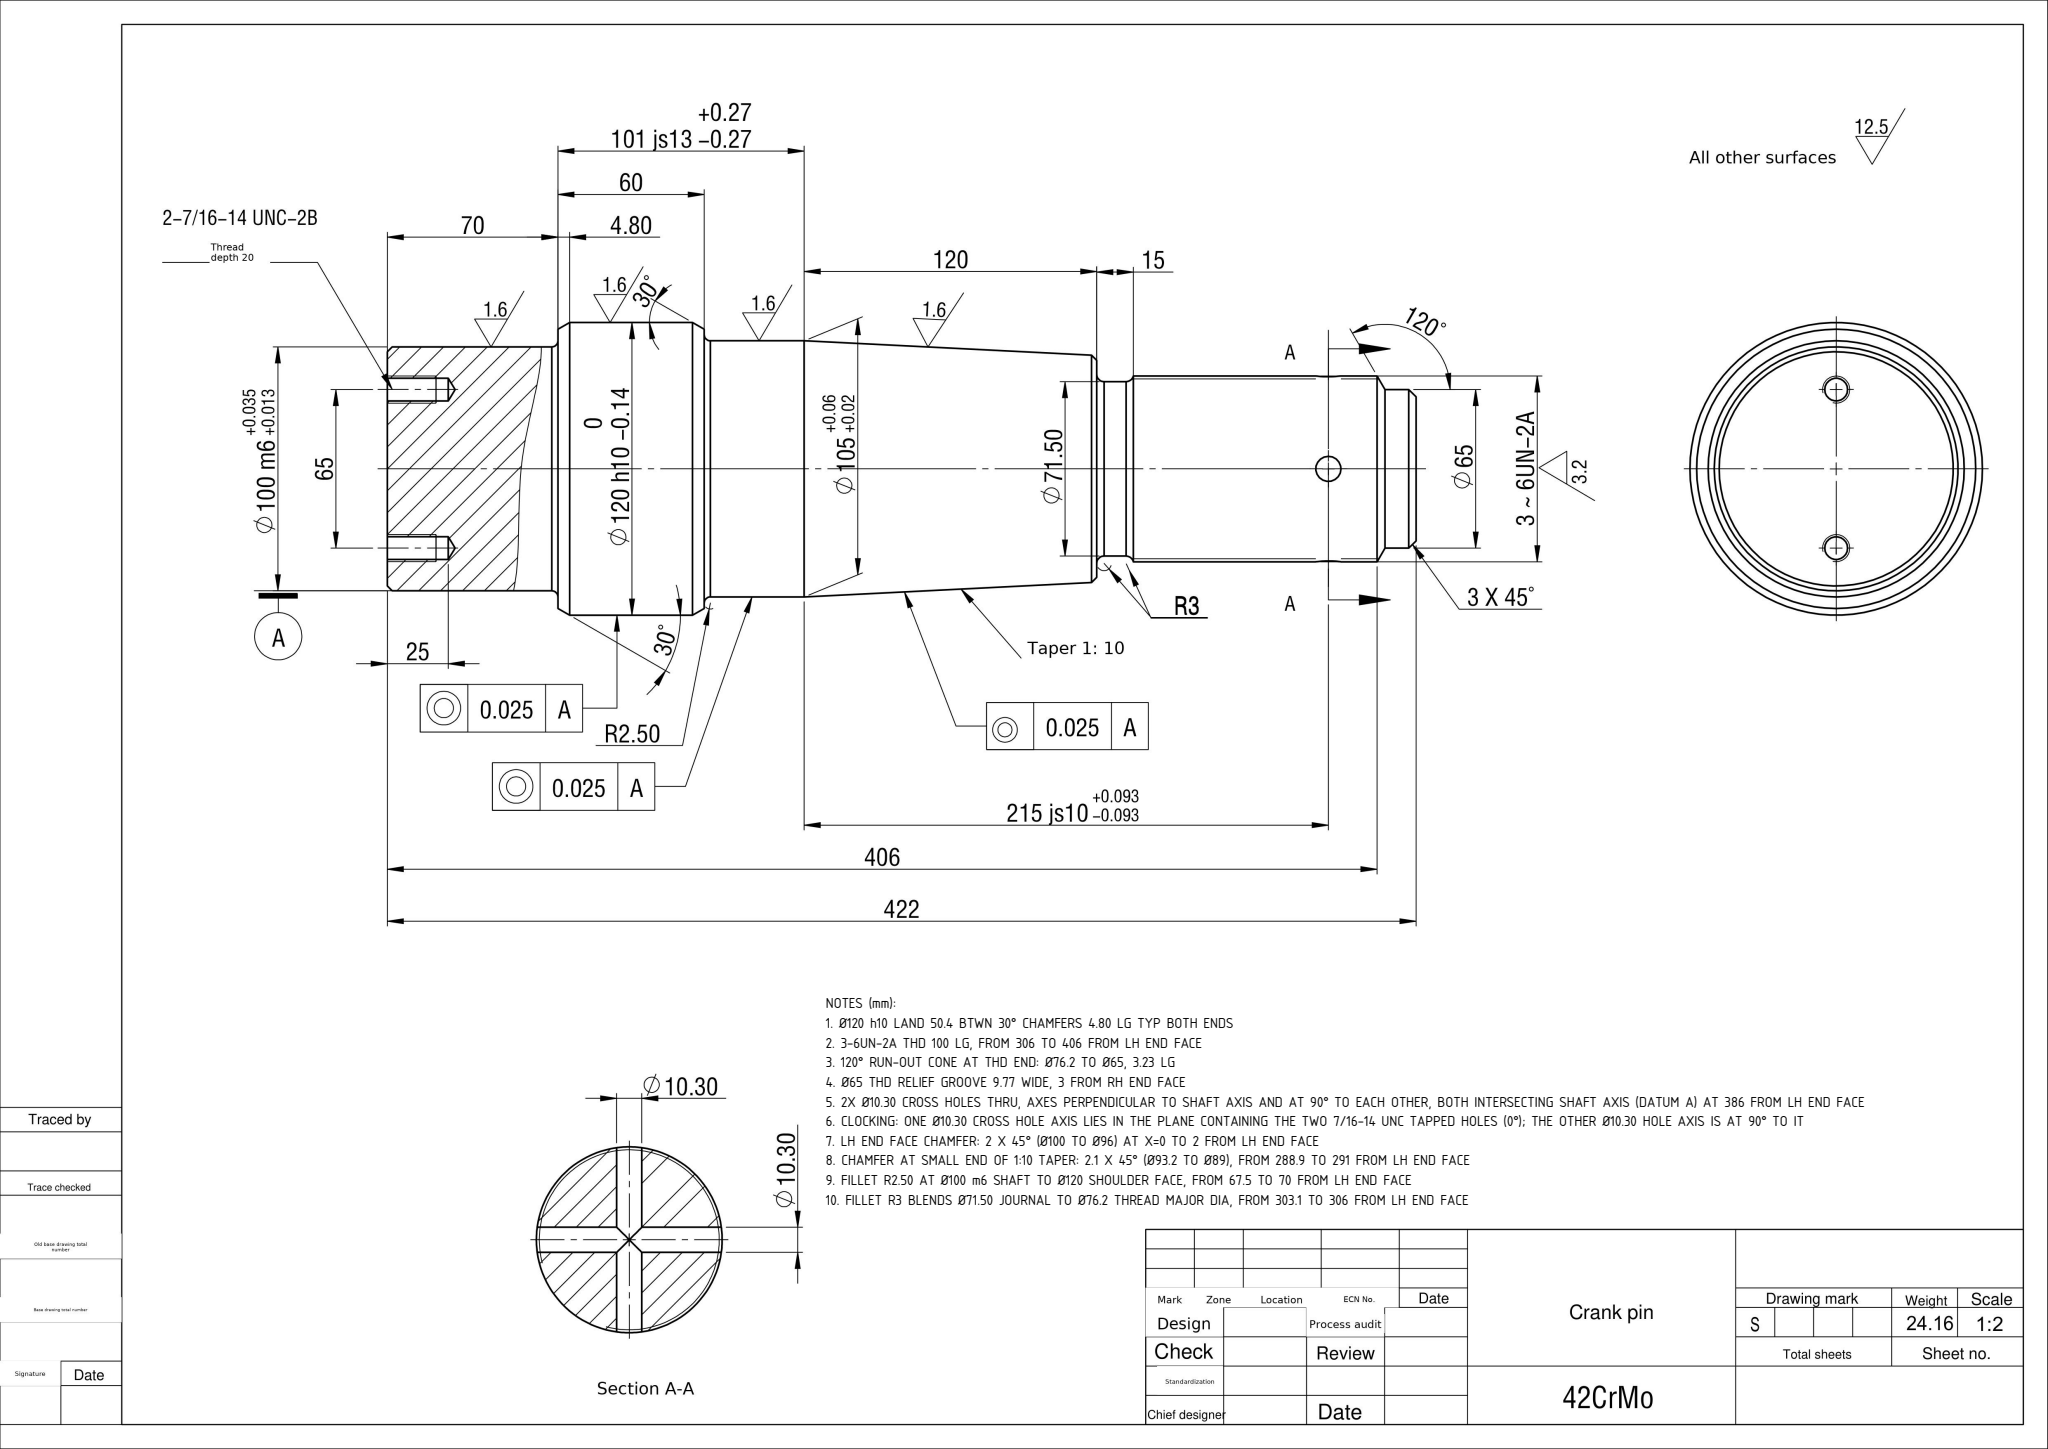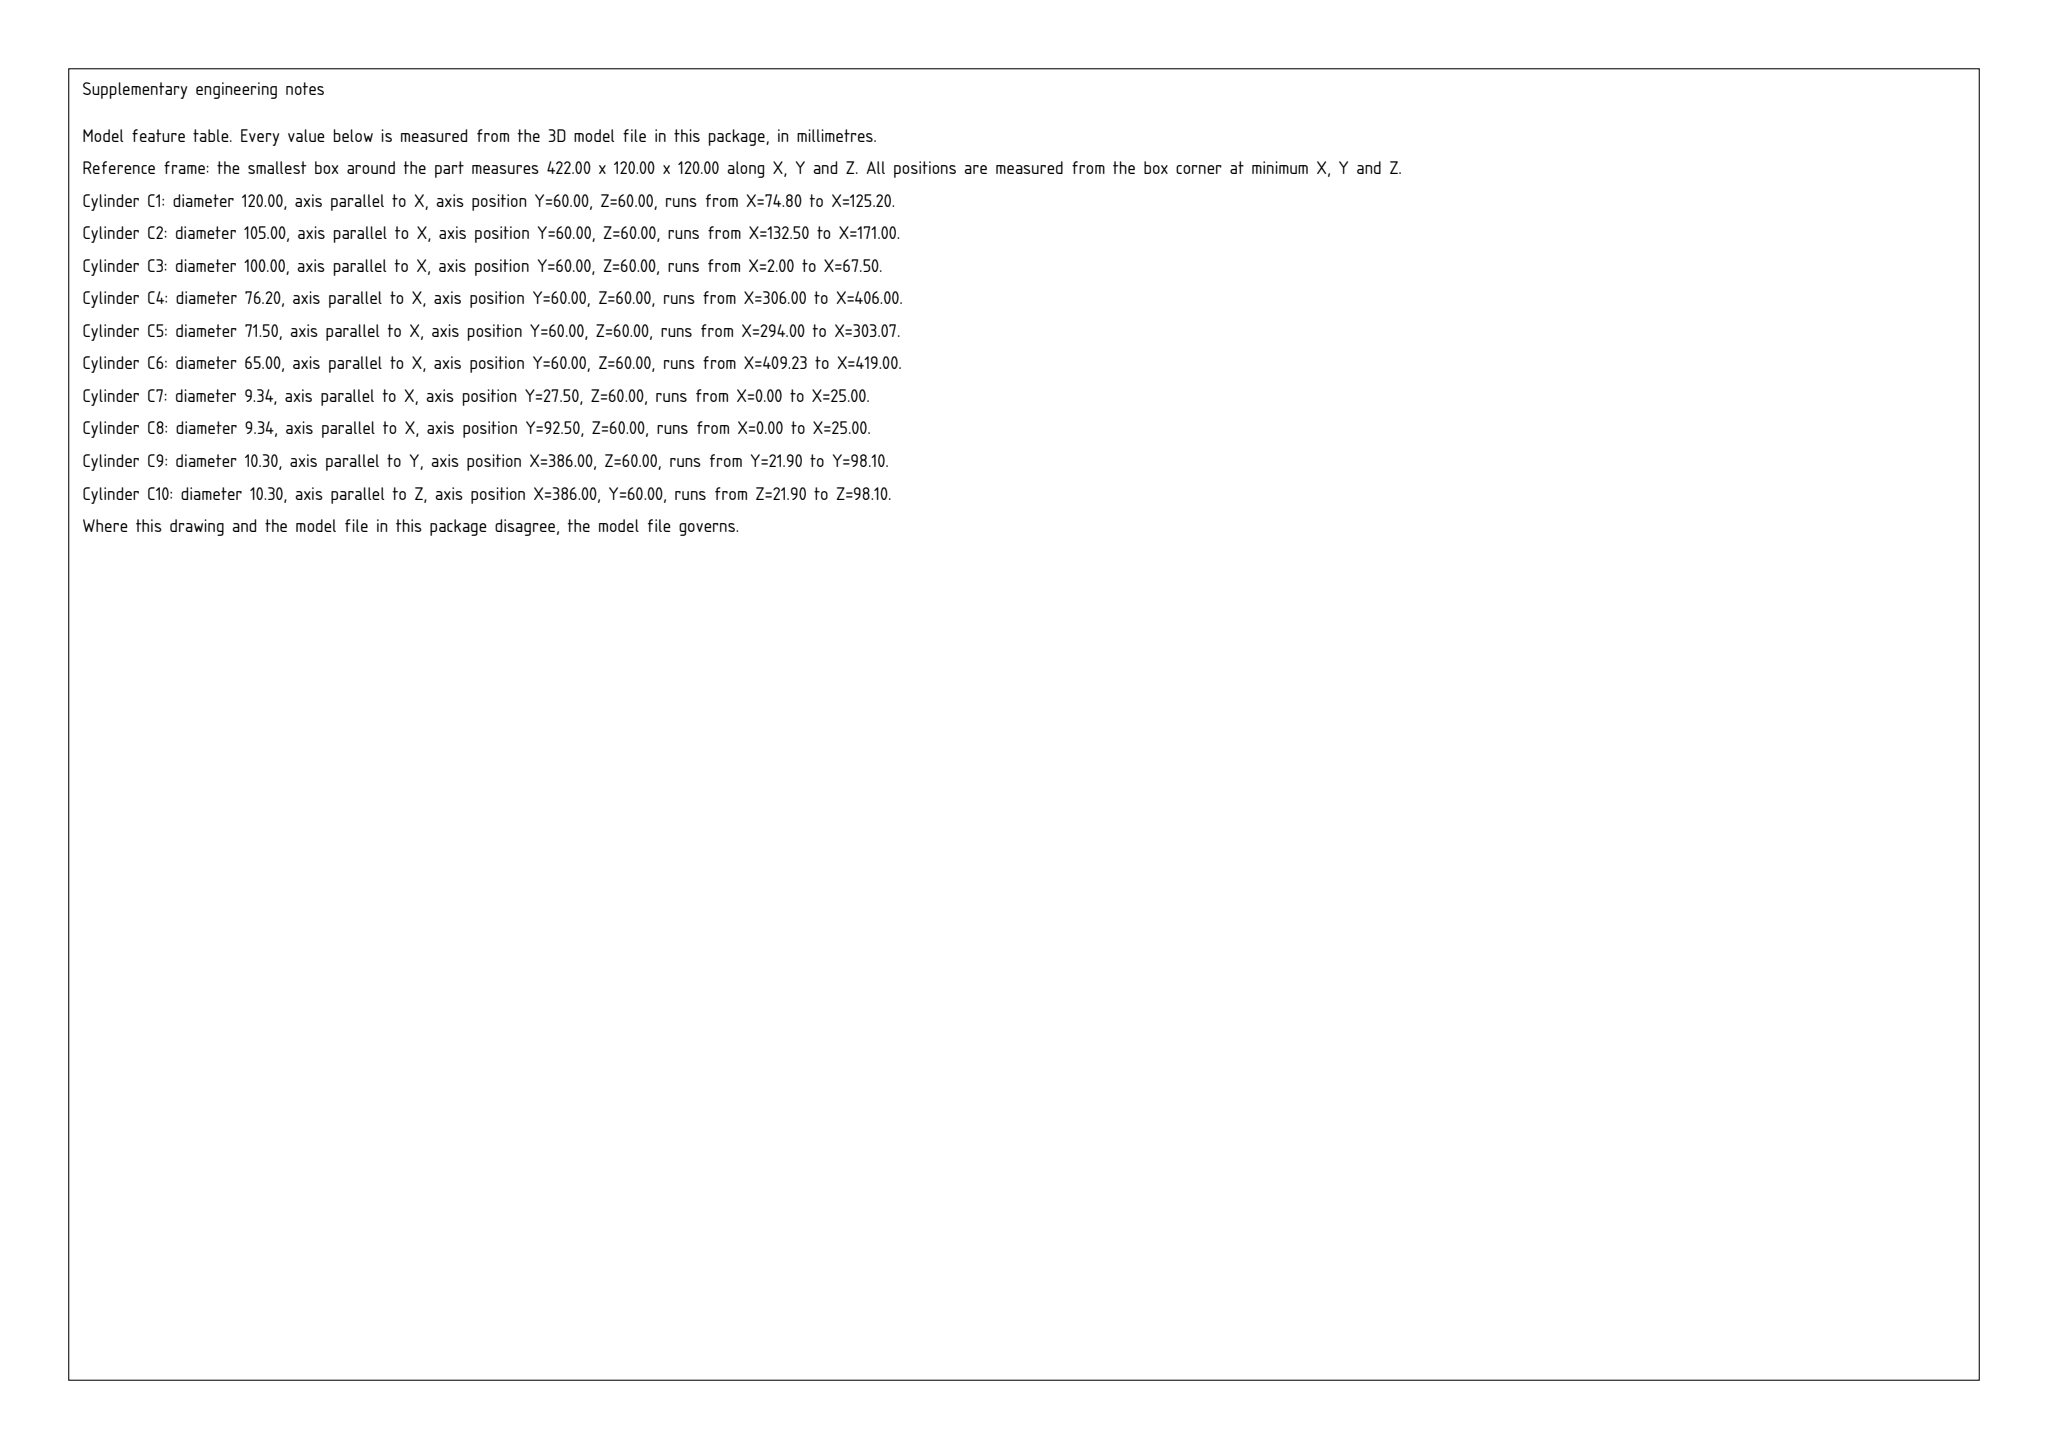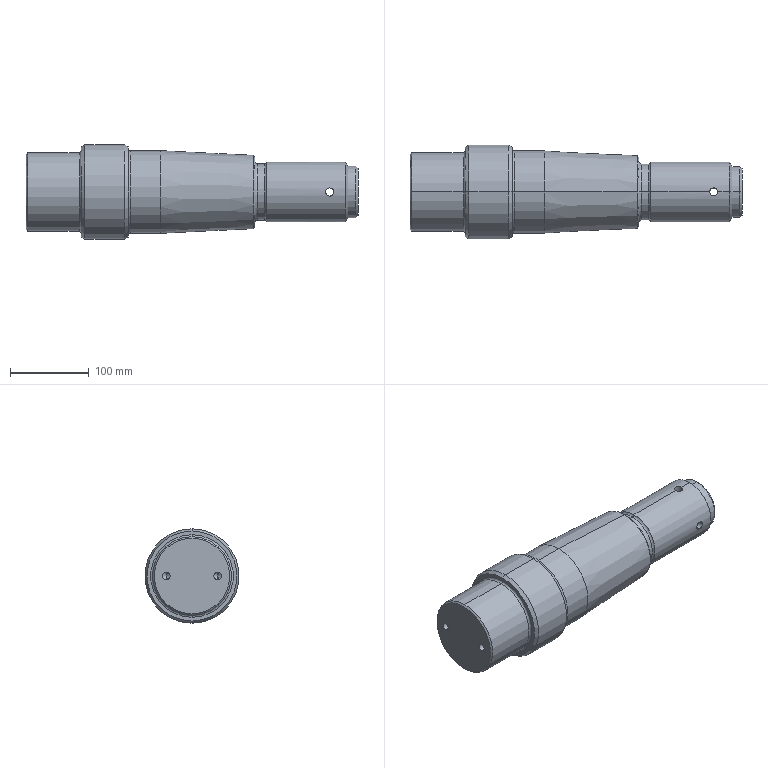Part | SolidWorks | mm | 1 solid | 55 faces | box 422 x 120 x 120 mm | volume 3058705 mm3 | cylinder 24 | cone 18 | torus 8 | plane 5 | commonest cylinder face diameters 10.3 x8 9.347 x4 65 x2 76.2 x2 71.5 x2 105 x2 120 x2 100 x2
Drawing notes:
Ø120 h10 LAND 50.4 BTWN 30° CHAMFERS 4.80 LG TYP BOTH ENDS | from the solid: 60° incl cone ref Ø120/Ø114.457; Ø120 cyl 50.4 = 60 - 2 x 4.80, boss x=70 to 130
3-6UN-2A THD 100 LG, FROM 306 TO 406 FROM LH END FACE | from the solid: Ø76.2 cyl, axis x, length 100, spans x=306 (end of 15 neck) to x=406; bbox x=0 at LH end face
120° RUN-OUT CONE AT THD END: Ø76.2 TO Ø65, 3.23 LG | from the solid: cone incl angle 120°, ref dia 65, joins Ø76.2 thd at x=406 to Ø65 groove at x=409.23
Ø65 THD RELIEF GROOVE 9.77 WIDE, 3 FROM RH END FACE | from the solid: Ø65 cyl length 9.77 (x=409.23 to 419), followed by 90° cone ref Ø65 (3x45 chamfer) to end face x=422
2X Ø10.30 CROSS HOLES THRU, AXES PERPENDICULAR TO SHAFT AXIS AND AT 90° TO EACH OTHER, BOTH INTERSECTING SHAFT AXIS (DATUM A) AT 386 FROM LH END FACE | from the solid: cylinders hole/bore Ø10.3 on y axis at [386,-,60] and Ø10.3 on z axis at [386,60,-], both spanning 21.9 to 98.1 (full 120 width)
CLOCKING: ONE Ø10.30 CROSS HOLE AXIS LIES IN THE PLANE CONTAINING THE TWO 7/16-14 UNC TAPPED HOLES (0°); THE OTHER Ø10.30 HOLE AXIS IS AT 90° TO IT | from the solid: tapped-hole cylinders Ø9.35 on x axis at y=27.5 and y=92.5, z=60 (line parallel to Y); Ø10.3 hole axes are along Y and along Z
LH END FACE CHAMFER: 2 X 45° (Ø100 TO Ø96) AT X=0 TO 2 FROM LH END FACE | from the solid: axis_planes x=0 extent y/z 12.0-108.0 (Ø96 face) with cylinder Ø100 starting at x=2.0
CHAMFER AT SMALL END OF 1:10 TAPER: 2.1 X 45° (Ø93.2 TO Ø89), FROM 288.9 TO 291 FROM LH END FACE | from the solid: cone included_angle 90.0, ref_dia 93.21, bbox_from x=288.9, size 2.1; axis_plane x=291 extent 15.5-104.5 (Ø89)
FILLET R2.50 AT Ø100 m6 SHAFT TO Ø120 SHOULDER FACE, FROM 67.5 TO 70 FROM LH END FACE | from the solid: torus minor_r 2.5 / major_r 52.5 (x2) between Ø100 cylinder ending at x=67.5 and plane x=70
FILLET R3 BLENDS Ø71.50 JOURNAL TO Ø76.2 THREAD MAJOR DIA, FROM 303.1 TO 306 FROM LH END FACE | from the solid: torus minor_r 3 / major_r 38.75 between Ø71.5 cylinder (to x=303.1) and Ø76.2 cylinder (from x=306)